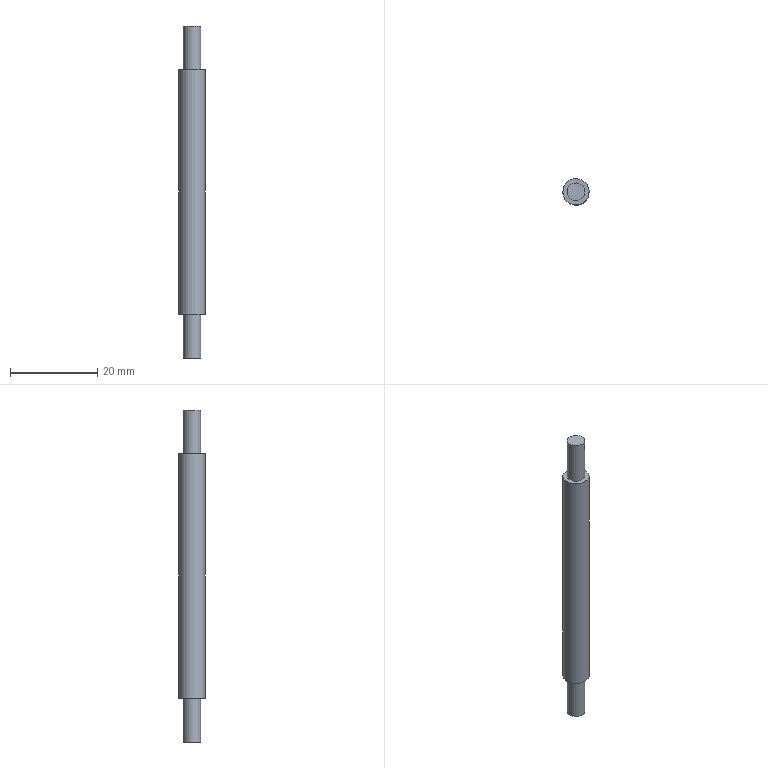Component | NX | 18B__27 | 1 solid | 7 faces | box 6 x 6 x 76 mm | volume 1835 mm3 | plane 4 | cylinder 3 | commonest cylinder face diameters 4 x2 6 x1
STEP:
#1=CARTESIAN_POINT('',(0.,0.,0.));
#2=DIRECTION('',(0.,0.,1.));
#3=DIRECTION('',(1.,0.,0.));
#4=AXIS2_PLACEMENT_3D('',#1,#2,#3);
#5=CARTESIAN_POINT('',(117.998,109.301,202.199));
#6=VERTEX_POINT('',#5);
#7=CARTESIAN_POINT('',(116.022,109.608,202.199));
#8=DIRECTION('',(0.,0.,1.));
#9=DIRECTION('',(0.9881,-0.1536,0.));
#10=AXIS2_PLACEMENT_3D('',#7,#8,#9);
#11=CIRCLE('',#10,2.);
#12=CARTESIAN_POINT('',(116.329,111.584,202.199));
#13=DIRECTION('',(0.,0.,-1.));
#14=DIRECTION('',(-0.9881,0.1536,0.));
#15=AXIS2_PLACEMENT_3D('',#12,#13,#14);
#16=PLANE('',#15);
#17=CARTESIAN_POINT('',(-2.,-2.));
#18=CARTESIAN_POINT('',(-2.,1.464));
#19=CARTESIAN_POINT('',(1.,-0.2679));
#20=CARTESIAN_POINT('',(4.,-2.));
#21=CARTESIAN_POINT('',(1.,-3.732));
#22=CARTESIAN_POINT('',(-2.,-5.464));
#23=CARTESIAN_POINT('',(-2.,-2.));
#24=(BOUNDED_CURVE()B_SPLINE_CURVE(2,(#17,#18,#19,#20,#21,#22,#23),.UNSPECIFIED.,.T.,.F.)B_SPLINE_CURVE_WITH_KNOTS((1,2,2,2,2,1),(-2.094,0.,2.094,4.189,6.283,8.378),.UNSPECIFIED.)CURVE()GEOMETRIC_REPRESENTATION_ITEM()RATIONAL_B_SPLINE_CURVE((1.,0.5,1.,0.5,1.,0.5,1.))REPRESENTATION_ITEM(''));
#25=(GEOMETRIC_REPRESENTATION_CONTEXT(2)PARAMETRIC_REPRESENTATION_CONTEXT()REPRESENTATION_CONTEXT('',''));
#26=DEFINITIONAL_REPRESENTATION('',(#24),#25);
#27=PCURVE('',#16,#26);
#28=CARTESIAN_POINT('',(116.022,109.608,136.199));
#29=DIRECTION('',(0.,0.,1.));
#30=DIRECTION('',(0.9881,-0.1536,0.));
#31=AXIS2_PLACEMENT_3D('',#28,#29,#30);
#32=CYLINDRICAL_SURFACE('',#31,2.);
#33=CARTESIAN_POINT('',(0.,66.));
#34=DIRECTION('',(1.,0.));
#35=VECTOR('',#34,1.);
#36=LINE('',#33,#35);
#37=(GEOMETRIC_REPRESENTATION_CONTEXT(2)PARAMETRIC_REPRESENTATION_CONTEXT()REPRESENTATION_CONTEXT('',''));
#38=DEFINITIONAL_REPRESENTATION('',(#36),#37);
#39=PCURVE('',#32,#38);
#40=SURFACE_CURVE('',#11,(#27,#39),.PCURVE_S1.);
#41=EDGE_CURVE('',#6,#6,#40,.T.);
#42=ORIENTED_EDGE('',*,*,#41,.T.);
#43=EDGE_LOOP('',(#42));
#44=FACE_BOUND('',#43,.T.);
#45=ADVANCED_FACE('',(#44),#16,.F.);
#46=CARTESIAN_POINT('',(117.998,109.301,126.199));
#47=VERTEX_POINT('',#46);
#48=CARTESIAN_POINT('',(116.022,109.608,126.199));
#49=DIRECTION('',(0.,0.,1.));
#50=DIRECTION('',(0.9881,-0.1536,0.));
#51=AXIS2_PLACEMENT_3D('',#48,#49,#50);
#52=CIRCLE('',#51,2.);
#53=CARTESIAN_POINT('',(116.022,109.608,126.199));
#54=DIRECTION('',(0.,0.,1.));
#55=DIRECTION('',(0.9881,-0.1536,0.));
#56=AXIS2_PLACEMENT_3D('',#53,#54,#55);
#57=PLANE('',#56);
#58=CARTESIAN_POINT('',(0.,0.));
#59=DIRECTION('',(1.,0.));
#60=AXIS2_PLACEMENT_2D('',#58,#59);
#61=CIRCLE('',#60,2.);
#62=(GEOMETRIC_REPRESENTATION_CONTEXT(2)PARAMETRIC_REPRESENTATION_CONTEXT()REPRESENTATION_CONTEXT('',''));
#63=DEFINITIONAL_REPRESENTATION('',(#61),#62);
#64=PCURVE('',#57,#63);
#65=CARTESIAN_POINT('',(116.022,109.608,136.199));
#66=DIRECTION('',(0.,0.,1.));
#67=DIRECTION('',(0.9881,-0.1536,0.));
#68=AXIS2_PLACEMENT_3D('',#65,#66,#67);
#69=CYLINDRICAL_SURFACE('',#68,2.);
#70=CARTESIAN_POINT('',(0.,-10.));
#71=DIRECTION('',(1.,0.));
#72=VECTOR('',#71,1.);
#73=LINE('',#70,#72);
#74=(GEOMETRIC_REPRESENTATION_CONTEXT(2)PARAMETRIC_REPRESENTATION_CONTEXT()REPRESENTATION_CONTEXT('',''));
#75=DEFINITIONAL_REPRESENTATION('',(#73),#74);
#76=PCURVE('',#69,#75);
#77=SURFACE_CURVE('',#52,(#64,#76),.PCURVE_S1.);
#78=EDGE_CURVE('',#47,#47,#77,.T.);
#79=ORIENTED_EDGE('',*,*,#78,.F.);
#80=EDGE_LOOP('',(#79));
#81=FACE_BOUND('',#80,.T.);
#82=ADVANCED_FACE('',(#81),#57,.F.);
#83=CARTESIAN_POINT('',(117.998,109.301,136.199));
#84=VERTEX_POINT('',#83);
#85=CARTESIAN_POINT('',(116.022,109.608,136.199));
#86=DIRECTION('',(0.,0.,1.));
#87=DIRECTION('',(0.9881,-0.1536,0.));
#88=AXIS2_PLACEMENT_3D('',#85,#86,#87);
#89=CIRCLE('',#88,2.);
#90=CARTESIAN_POINT('',(0.,0.));
#91=DIRECTION('',(1.,0.));
#92=VECTOR('',#91,1.);
#93=LINE('',#90,#92);
#94=(GEOMETRIC_REPRESENTATION_CONTEXT(2)PARAMETRIC_REPRESENTATION_CONTEXT()REPRESENTATION_CONTEXT('',''));
#95=DEFINITIONAL_REPRESENTATION('',(#93),#94);
#96=PCURVE('',#69,#95);
#97=CARTESIAN_POINT('',(116.329,111.584,136.199));
#98=DIRECTION('',(0.,0.,1.));
#99=DIRECTION('',(0.9881,-0.1536,0.));
#100=AXIS2_PLACEMENT_3D('',#97,#98,#99);
#101=PLANE('',#100);
#102=CARTESIAN_POINT('',(0.,-2.));
#103=DIRECTION('',(1.,0.));
#104=AXIS2_PLACEMENT_2D('',#102,#103);
#105=CIRCLE('',#104,2.);
#106=(GEOMETRIC_REPRESENTATION_CONTEXT(2)PARAMETRIC_REPRESENTATION_CONTEXT()REPRESENTATION_CONTEXT('',''));
#107=DEFINITIONAL_REPRESENTATION('',(#105),#106);
#108=PCURVE('',#101,#107);
#109=SURFACE_CURVE('',#89,(#96,#108),.PCURVE_S1.);
#110=EDGE_CURVE('',#84,#84,#109,.T.);
#111=ORIENTED_EDGE('',*,*,#110,.F.);
#112=CARTESIAN_POINT('',(117.998,109.301,126.199));
#113=CARTESIAN_POINT('',(117.998,109.301,136.199));
#114=B_SPLINE_CURVE_WITH_KNOTS('',1,(#112,#113),.UNSPECIFIED.,.F.,.F.,(2,2),(-10.,0.),.PIECEWISE_BEZIER_KNOTS.);
#115=CARTESIAN_POINT('',(0.,0.));
#116=DIRECTION('',(0.,1.));
#117=VECTOR('',#116,1.);
#118=LINE('',#115,#117);
#119=(GEOMETRIC_REPRESENTATION_CONTEXT(2)PARAMETRIC_REPRESENTATION_CONTEXT()REPRESENTATION_CONTEXT('',''));
#120=DEFINITIONAL_REPRESENTATION('',(#118),#119);
#121=PCURVE('',#69,#120);
#122=CARTESIAN_POINT('',(6.283,0.));
#123=DIRECTION('',(0.,1.));
#124=VECTOR('',#123,1.);
#125=LINE('',#122,#124);
#126=(GEOMETRIC_REPRESENTATION_CONTEXT(2)PARAMETRIC_REPRESENTATION_CONTEXT()REPRESENTATION_CONTEXT('',''));
#127=DEFINITIONAL_REPRESENTATION('',(#125),#126);
#128=PCURVE('',#69,#127);
#129=SEAM_CURVE('',#114,(#121,#128),.PCURVE_S1.);
#130=EDGE_CURVE('',#47,#84,#129,.T.);
#131=ORIENTED_EDGE('',*,*,#130,.F.);
#132=ORIENTED_EDGE('',*,*,#78,.T.);
#133=ORIENTED_EDGE('',*,*,#130,.T.);
#134=EDGE_LOOP('',(#111,#131,#132,#133));
#135=FACE_BOUND('',#134,.T.);
#136=ADVANCED_FACE('',(#135),#69,.T.);
#137=CARTESIAN_POINT('',(118.987,109.147,136.199));
#138=VERTEX_POINT('',#137);
#139=CARTESIAN_POINT('',(116.022,109.608,136.199));
#140=DIRECTION('',(0.,0.,1.));
#141=DIRECTION('',(0.9881,-0.1536,0.));
#142=AXIS2_PLACEMENT_3D('',#139,#140,#141);
#143=CIRCLE('',#142,3.);
#144=CARTESIAN_POINT('',(0.,-2.));
#145=DIRECTION('',(1.,0.));
#146=AXIS2_PLACEMENT_2D('',#144,#145);
#147=CIRCLE('',#146,3.);
#148=(GEOMETRIC_REPRESENTATION_CONTEXT(2)PARAMETRIC_REPRESENTATION_CONTEXT()REPRESENTATION_CONTEXT('',''));
#149=DEFINITIONAL_REPRESENTATION('',(#147),#148);
#150=PCURVE('',#101,#149);
#151=CARTESIAN_POINT('',(116.022,109.608,136.199));
#152=DIRECTION('',(0.,0.,1.));
#153=DIRECTION('',(0.9881,-0.1536,0.));
#154=AXIS2_PLACEMENT_3D('',#151,#152,#153);
#155=CYLINDRICAL_SURFACE('',#154,3.);
#156=CARTESIAN_POINT('',(0.,0.));
#157=DIRECTION('',(1.,0.));
#158=VECTOR('',#157,1.);
#159=LINE('',#156,#158);
#160=(GEOMETRIC_REPRESENTATION_CONTEXT(2)PARAMETRIC_REPRESENTATION_CONTEXT()REPRESENTATION_CONTEXT('',''));
#161=DEFINITIONAL_REPRESENTATION('',(#159),#160);
#162=PCURVE('',#155,#161);
#163=SURFACE_CURVE('',#143,(#150,#162),.PCURVE_S1.);
#164=EDGE_CURVE('',#138,#138,#163,.T.);
#165=ORIENTED_EDGE('',*,*,#164,.F.);
#166=EDGE_LOOP('',(#165));
#167=FACE_BOUND('',#166,.T.);
#168=ORIENTED_EDGE('',*,*,#110,.T.);
#169=EDGE_LOOP('',(#168));
#170=FACE_BOUND('',#169,.T.);
#171=ADVANCED_FACE('',(#167,#170),#101,.F.);
#172=CARTESIAN_POINT('',(118.987,109.147,192.199));
#173=VERTEX_POINT('',#172);
#174=CARTESIAN_POINT('',(116.022,109.608,192.199));
#175=DIRECTION('',(0.,0.,1.));
#176=DIRECTION('',(0.9881,-0.1536,0.));
#177=AXIS2_PLACEMENT_3D('',#174,#175,#176);
#178=CIRCLE('',#177,3.);
#179=CARTESIAN_POINT('',(0.,56.));
#180=DIRECTION('',(1.,0.));
#181=VECTOR('',#180,1.);
#182=LINE('',#179,#181);
#183=(GEOMETRIC_REPRESENTATION_CONTEXT(2)PARAMETRIC_REPRESENTATION_CONTEXT()REPRESENTATION_CONTEXT('',''));
#184=DEFINITIONAL_REPRESENTATION('',(#182),#183);
#185=PCURVE('',#155,#184);
#186=CARTESIAN_POINT('',(116.483,112.573,192.199));
#187=DIRECTION('',(0.,0.,-1.));
#188=DIRECTION('',(-0.9881,0.1536,0.));
#189=AXIS2_PLACEMENT_3D('',#186,#187,#188);
#190=PLANE('',#189);
#191=CARTESIAN_POINT('',(-3.,-3.));
#192=CARTESIAN_POINT('',(-3.,2.196));
#193=CARTESIAN_POINT('',(1.5,-0.4019));
#194=CARTESIAN_POINT('',(6.,-3.));
#195=CARTESIAN_POINT('',(1.5,-5.598));
#196=CARTESIAN_POINT('',(-3.,-8.196));
#197=CARTESIAN_POINT('',(-3.,-3.));
#198=(BOUNDED_CURVE()B_SPLINE_CURVE(2,(#191,#192,#193,#194,#195,#196,#197),.UNSPECIFIED.,.T.,.F.)B_SPLINE_CURVE_WITH_KNOTS((1,2,2,2,2,1),(-2.094,0.,2.094,4.189,6.283,8.378),.UNSPECIFIED.)CURVE()GEOMETRIC_REPRESENTATION_ITEM()RATIONAL_B_SPLINE_CURVE((1.,0.5,1.,0.5,1.,0.5,1.))REPRESENTATION_ITEM(''));
#199=(GEOMETRIC_REPRESENTATION_CONTEXT(2)PARAMETRIC_REPRESENTATION_CONTEXT()REPRESENTATION_CONTEXT('',''));
#200=DEFINITIONAL_REPRESENTATION('',(#198),#199);
#201=PCURVE('',#190,#200);
#202=SURFACE_CURVE('',#178,(#185,#201),.PCURVE_S1.);
#203=EDGE_CURVE('',#173,#173,#202,.T.);
#204=ORIENTED_EDGE('',*,*,#203,.F.);
#205=CARTESIAN_POINT('',(118.987,109.147,136.199));
#206=CARTESIAN_POINT('',(118.987,109.147,192.199));
#207=B_SPLINE_CURVE_WITH_KNOTS('',1,(#205,#206),.UNSPECIFIED.,.F.,.F.,(2,2),(0.,56.),.PIECEWISE_BEZIER_KNOTS.);
#208=CARTESIAN_POINT('',(0.,0.));
#209=DIRECTION('',(0.,1.));
#210=VECTOR('',#209,1.);
#211=LINE('',#208,#210);
#212=(GEOMETRIC_REPRESENTATION_CONTEXT(2)PARAMETRIC_REPRESENTATION_CONTEXT()REPRESENTATION_CONTEXT('',''));
#213=DEFINITIONAL_REPRESENTATION('',(#211),#212);
#214=PCURVE('',#155,#213);
#215=CARTESIAN_POINT('',(6.283,0.));
#216=DIRECTION('',(0.,1.));
#217=VECTOR('',#216,1.);
#218=LINE('',#215,#217);
#219=(GEOMETRIC_REPRESENTATION_CONTEXT(2)PARAMETRIC_REPRESENTATION_CONTEXT()REPRESENTATION_CONTEXT('',''));
#220=DEFINITIONAL_REPRESENTATION('',(#218),#219);
#221=PCURVE('',#155,#220);
#222=SEAM_CURVE('',#207,(#214,#221),.PCURVE_S1.);
#223=EDGE_CURVE('',#138,#173,#222,.T.);
#224=ORIENTED_EDGE('',*,*,#223,.F.);
#225=ORIENTED_EDGE('',*,*,#164,.T.);
#226=ORIENTED_EDGE('',*,*,#223,.T.);
#227=EDGE_LOOP('',(#204,#224,#225,#226));
#228=FACE_BOUND('',#227,.T.);
#229=ADVANCED_FACE('',(#228),#155,.T.);
#230=CARTESIAN_POINT('',(117.998,109.301,192.199));
#231=VERTEX_POINT('',#230);
#232=CARTESIAN_POINT('',(116.022,109.608,192.199));
#233=DIRECTION('',(0.,0.,1.));
#234=DIRECTION('',(0.9881,-0.1536,0.));
#235=AXIS2_PLACEMENT_3D('',#232,#233,#234);
#236=CIRCLE('',#235,2.);
#237=CARTESIAN_POINT('',(-2.,-3.));
#238=CARTESIAN_POINT('',(-2.,0.4641));
#239=CARTESIAN_POINT('',(1.,-1.268));
#240=CARTESIAN_POINT('',(4.,-3.));
#241=CARTESIAN_POINT('',(1.,-4.732));
#242=CARTESIAN_POINT('',(-2.,-6.464));
#243=CARTESIAN_POINT('',(-2.,-3.));
#244=(BOUNDED_CURVE()B_SPLINE_CURVE(2,(#237,#238,#239,#240,#241,#242,#243),.UNSPECIFIED.,.T.,.F.)B_SPLINE_CURVE_WITH_KNOTS((1,2,2,2,2,1),(-2.094,0.,2.094,4.189,6.283,8.378),.UNSPECIFIED.)CURVE()GEOMETRIC_REPRESENTATION_ITEM()RATIONAL_B_SPLINE_CURVE((1.,0.5,1.,0.5,1.,0.5,1.))REPRESENTATION_ITEM(''));
#245=(GEOMETRIC_REPRESENTATION_CONTEXT(2)PARAMETRIC_REPRESENTATION_CONTEXT()REPRESENTATION_CONTEXT('',''));
#246=DEFINITIONAL_REPRESENTATION('',(#244),#245);
#247=PCURVE('',#190,#246);
#248=CARTESIAN_POINT('',(0.,56.));
#249=DIRECTION('',(1.,0.));
#250=VECTOR('',#249,1.);
#251=LINE('',#248,#250);
#252=(GEOMETRIC_REPRESENTATION_CONTEXT(2)PARAMETRIC_REPRESENTATION_CONTEXT()REPRESENTATION_CONTEXT('',''));
#253=DEFINITIONAL_REPRESENTATION('',(#251),#252);
#254=PCURVE('',#32,#253);
#255=SURFACE_CURVE('',#236,(#247,#254),.PCURVE_S1.);
#256=EDGE_CURVE('',#231,#231,#255,.T.);
#257=ORIENTED_EDGE('',*,*,#256,.F.);
#258=EDGE_LOOP('',(#257));
#259=FACE_BOUND('',#258,.T.);
#260=ORIENTED_EDGE('',*,*,#203,.T.);
#261=EDGE_LOOP('',(#260));
#262=FACE_BOUND('',#261,.T.);
#263=ADVANCED_FACE('',(#259,#262),#190,.F.);
#264=ORIENTED_EDGE('',*,*,#41,.F.);
#265=CARTESIAN_POINT('',(117.998,109.301,192.199));
#266=CARTESIAN_POINT('',(117.998,109.301,202.199));
#267=B_SPLINE_CURVE_WITH_KNOTS('',1,(#265,#266),.UNSPECIFIED.,.F.,.F.,(2,2),(56.,66.),.PIECEWISE_BEZIER_KNOTS.);
#268=CARTESIAN_POINT('',(0.,0.));
#269=DIRECTION('',(0.,1.));
#270=VECTOR('',#269,1.);
#271=LINE('',#268,#270);
#272=(GEOMETRIC_REPRESENTATION_CONTEXT(2)PARAMETRIC_REPRESENTATION_CONTEXT()REPRESENTATION_CONTEXT('',''));
#273=DEFINITIONAL_REPRESENTATION('',(#271),#272);
#274=PCURVE('',#32,#273);
#275=CARTESIAN_POINT('',(6.283,0.));
#276=DIRECTION('',(0.,1.));
#277=VECTOR('',#276,1.);
#278=LINE('',#275,#277);
#279=(GEOMETRIC_REPRESENTATION_CONTEXT(2)PARAMETRIC_REPRESENTATION_CONTEXT()REPRESENTATION_CONTEXT('',''));
#280=DEFINITIONAL_REPRESENTATION('',(#278),#279);
#281=PCURVE('',#32,#280);
#282=SEAM_CURVE('',#267,(#274,#281),.PCURVE_S1.);
#283=EDGE_CURVE('',#231,#6,#282,.T.);
#284=ORIENTED_EDGE('',*,*,#283,.F.);
#285=ORIENTED_EDGE('',*,*,#256,.T.);
#286=ORIENTED_EDGE('',*,*,#283,.T.);
#287=EDGE_LOOP('',(#264,#284,#285,#286));
#288=FACE_BOUND('',#287,.T.);
#289=ADVANCED_FACE('',(#288),#32,.T.);
#290=CLOSED_SHELL('',(#45,#82,#136,#171,#229,#263,#289));
#291=MANIFOLD_SOLID_BREP('',#290);
#292=(LENGTH_UNIT()NAMED_UNIT(*)SI_UNIT(.MILLI.,.METRE.));
#293=UNCERTAINTY_MEASURE_WITH_UNIT(LENGTH_MEASURE(0.00001),#292,'','');
#294=(NAMED_UNIT(*)PLANE_ANGLE_UNIT()SI_UNIT($,.RADIAN.));
#295=(NAMED_UNIT(*)SI_UNIT($,.STERADIAN.)SOLID_ANGLE_UNIT());
#296=(GEOMETRIC_REPRESENTATION_CONTEXT(3)GLOBAL_UNCERTAINTY_ASSIGNED_CONTEXT((#293))GLOBAL_UNIT_ASSIGNED_CONTEXT((#292,#294,#295))REPRESENTATION_CONTEXT('',''));
#297=ADVANCED_BREP_SHAPE_REPRESENTATION('',(#4,#291),#296);